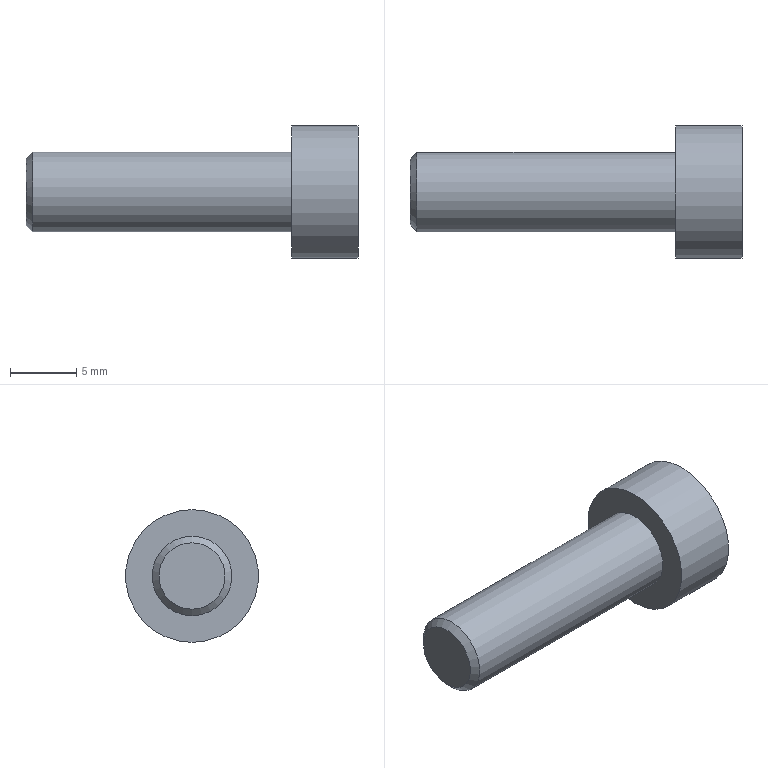Component | NX | BOLT_2 | 1 solid | 19 faces | volume 833 mm3 | plane 10 | cylinder 8 | cone 1 | commonest cylinder face diameters 4 x6 6 x1 10 x1